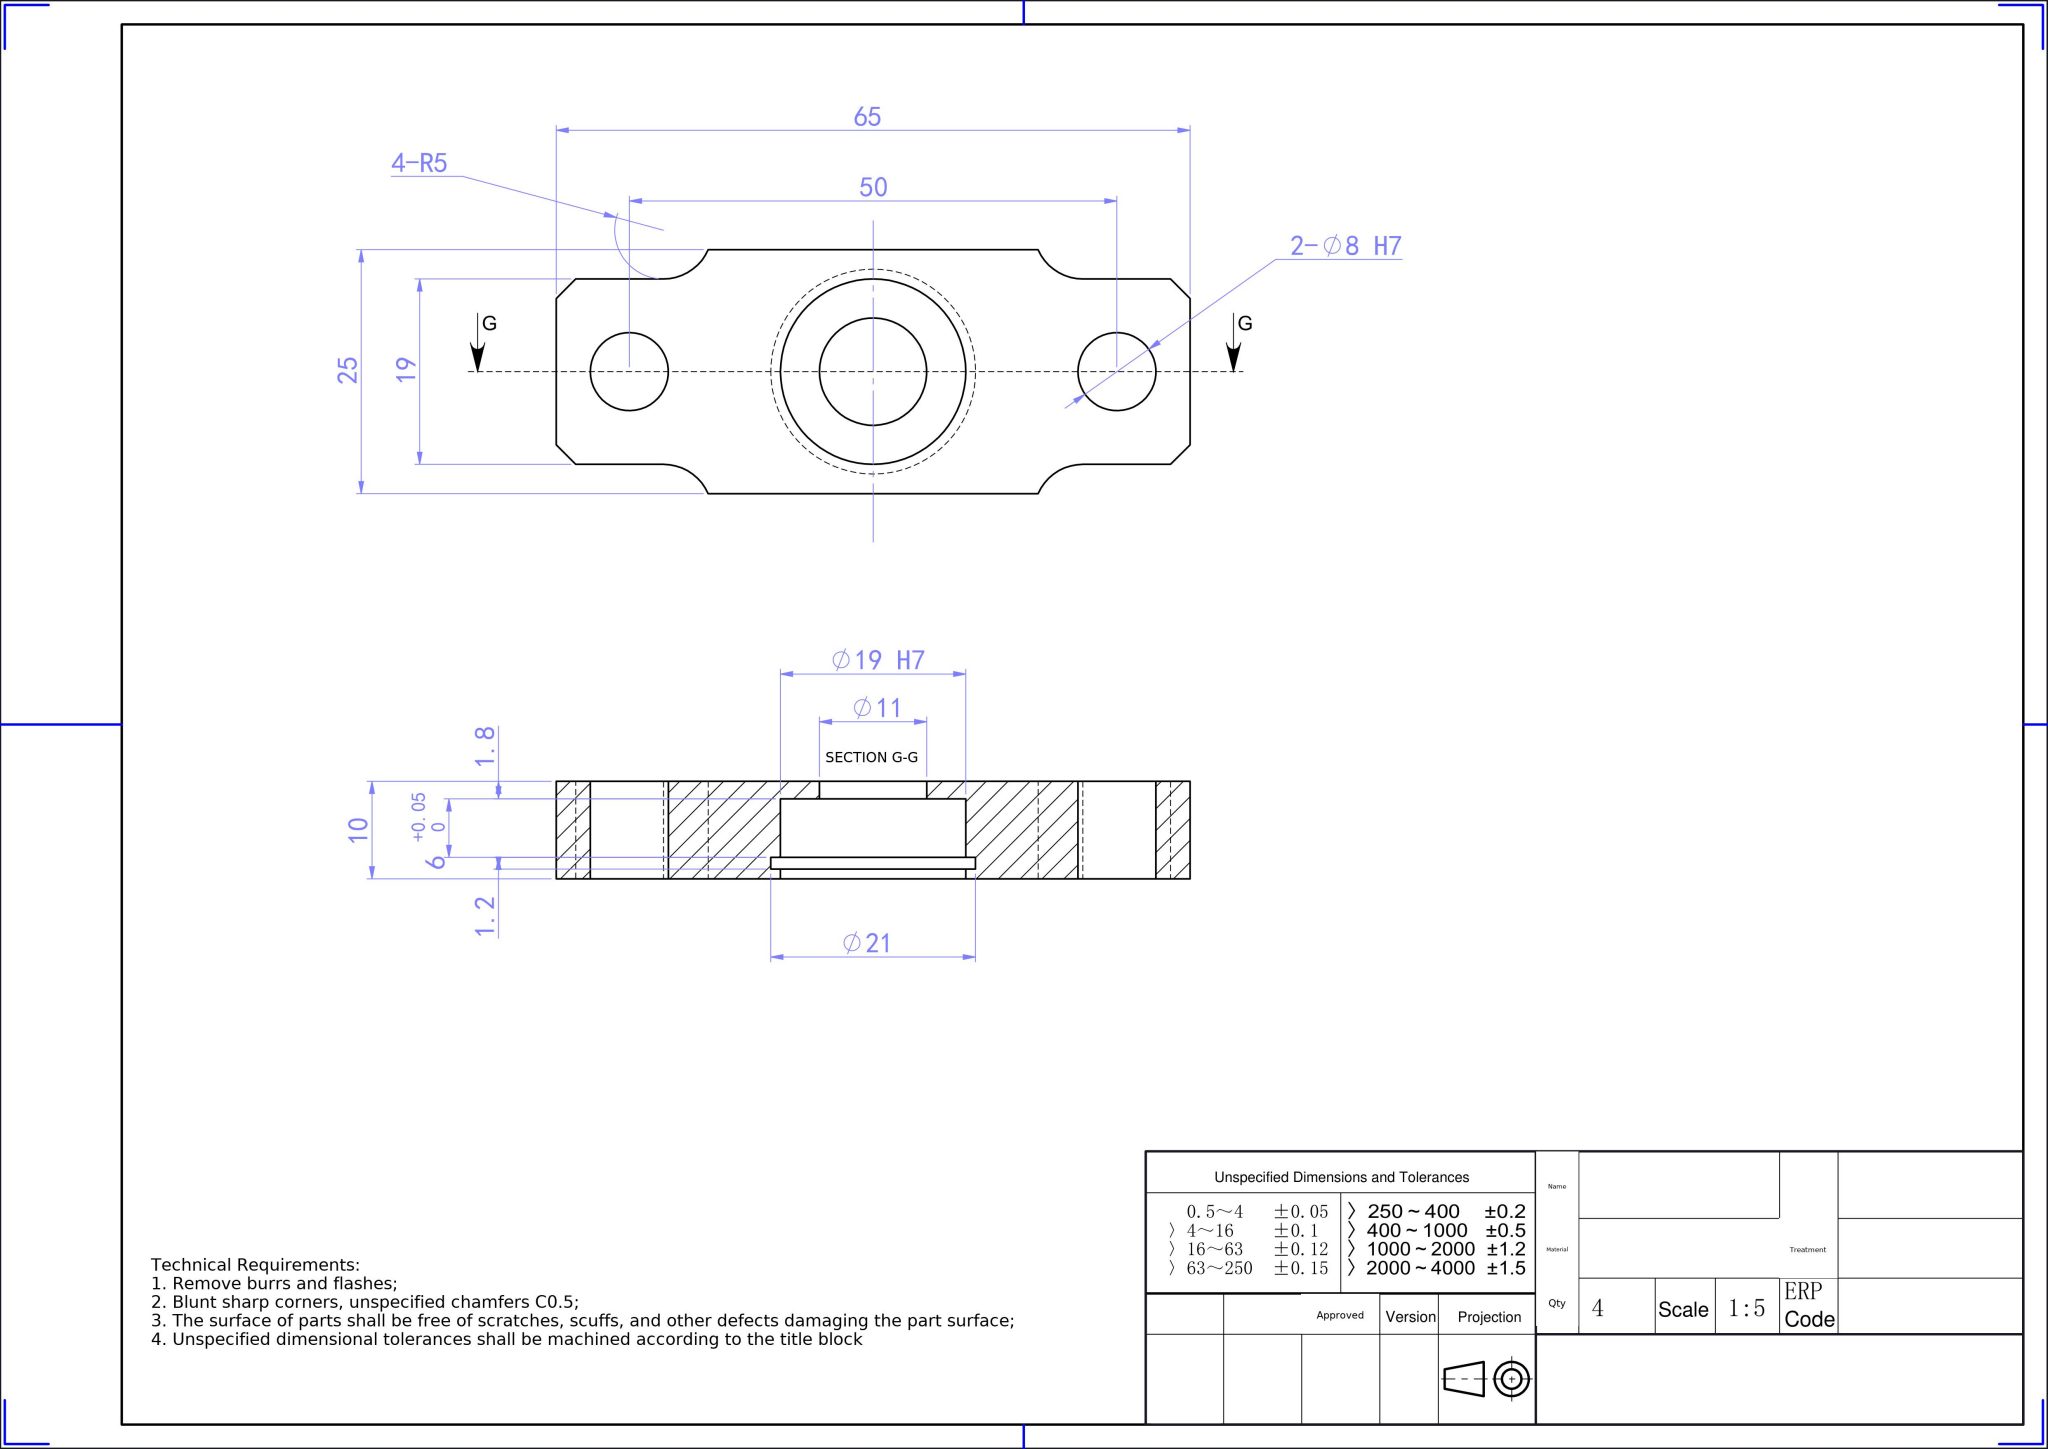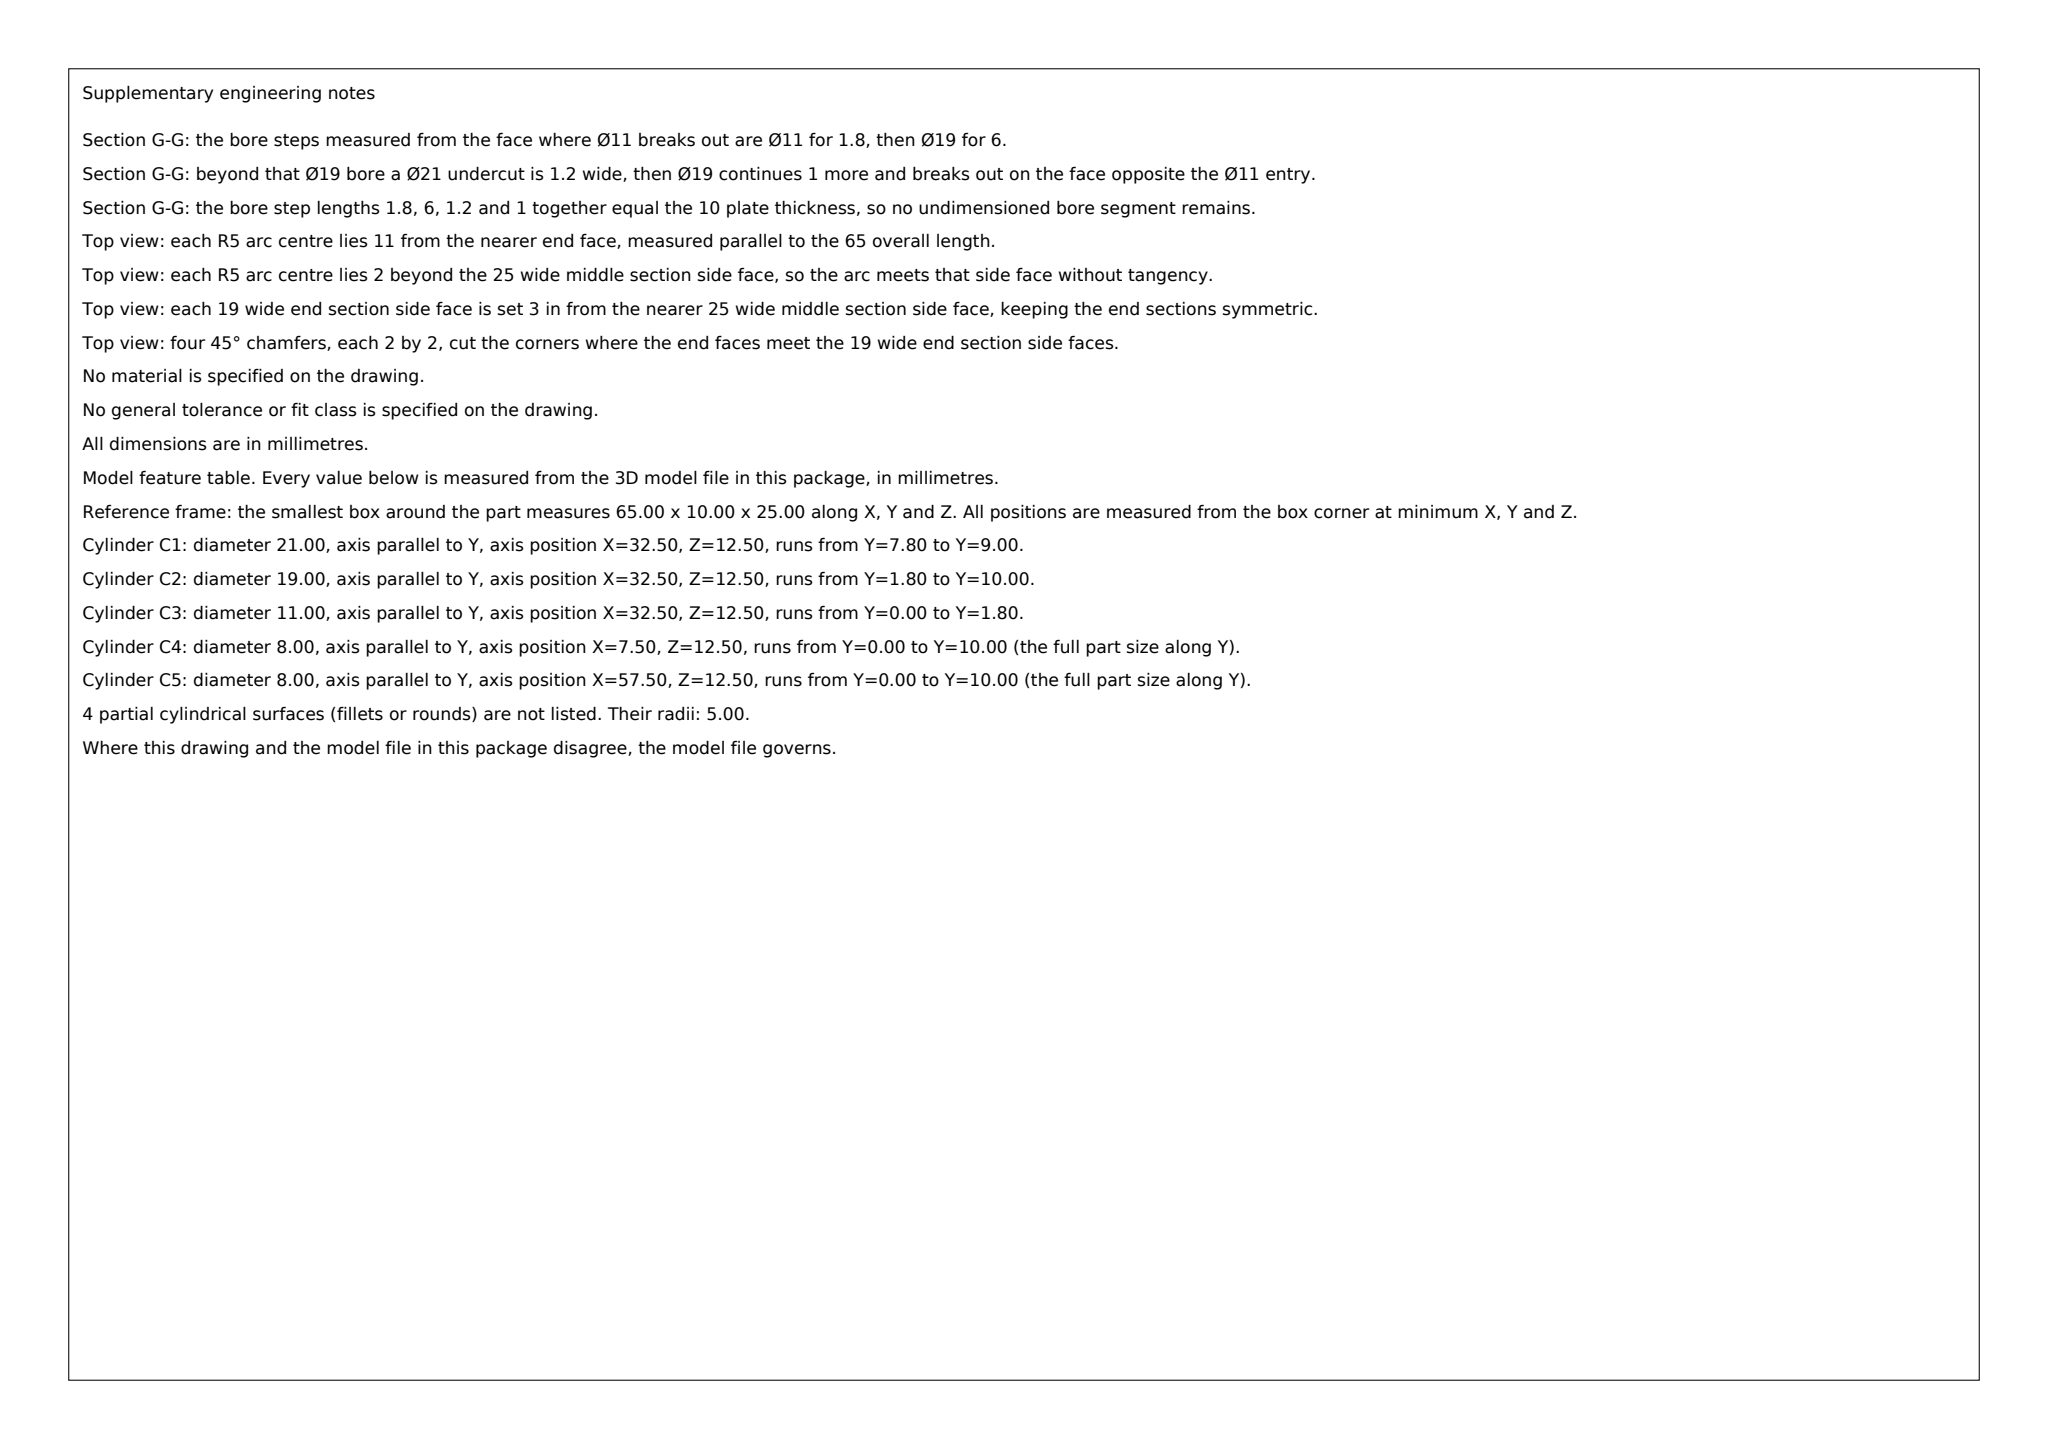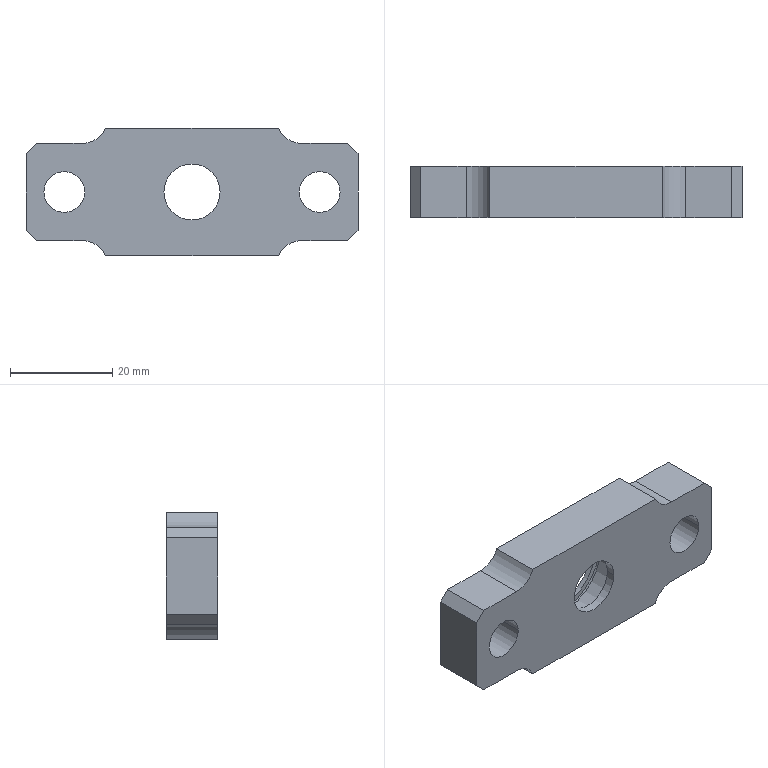Part | SolidWorks | mm | 1 solid | 33 faces | box 65 x 10 x 25 mm | volume 10877 mm3 | plane 17 | cylinder 16 | commonest cylinder face diameters 8 x4 19 x4 10 x4 11 x2 21 x2
Drawing notes:
4-R5 ARC CTRS 11 FROM EA END, 43 APART, ON Ø19 H7 C/L | from the solid: R5 corner cyl dia10 axes at x=11 & x=54 (bbox x=0..65); 65-54=11, 54-11=43; z=-2/27 => tangent to 19 wide flats about z=12.5
build123d program:
from build123d import *

# Parameters (mm, degrees)
SKETCH1_W      = 65
SKETCH1_H      = 10
EXTRUDE1_DEPTH = 25
CHAMFER1_SIZE  = 2
SKETCH11_R     = 4
EXTRUDE3_DEPTH = 18
EXTRUDE4_DEPTH = 18
CHAMFER2_SIZE  = 2


with BuildPart() as part:
    # Sketch1 → Extrude1 (new body)
    with BuildSketch(Plane.XY):
        with Locations((-11.635, 36.458)):
            Rectangle(SKETCH1_W, SKETCH1_H)
    extrude(amount=EXTRUDE1_DEPTH)

    # Chamfer1
    chamfer1_edges = [part.edges().sort_by_distance(p)[0] for p in [
        (20.865, 36.458, 25),
        (-44.135, 36.458, 25),
        (20.865, 36.458, 0),
        (-44.135, 36.458, 0),
    ]]
    chamfer(chamfer1_edges, length=CHAMFER1_SIZE)

    # Sketch9 → Cut-Revolve1 (revolve, cut)
    with BuildSketch(Plane(origin=(0, 0, 12.5), x_dir=(-1, 0, 0), z_dir=(0, 0, -1))):
        Polygon((21.135, 40.458), (22.135, 40.458), (22.135, 39.258), (21.135, 39.258), (21.135, 33.258), (17.135, 33.258), (17.135, 31.458), (11.635, 31.458), (11.635, 41.458), (21.135, 41.458), align=None)
    revolve(axis=Axis((-11.635, 41.458, 12.5), (0, -1, 0)), mode=Mode.SUBTRACT)

    # Sketch11 → Extrude3 (cut)
    with BuildSketch(Plane(origin=(0, 41.458, 0), x_dir=(-1, 0, 0), z_dir=(0, 1, 0))):
        with Locations((36.635, 12.5)):
            Circle(SKETCH11_R)
        with Locations((-13.365, 12.5)):
            Circle(SKETCH11_R)
    extrude(amount=-EXTRUDE3_DEPTH, mode=Mode.SUBTRACT)

    # Sketch12 → Extrude4 (cut)
    with BuildSketch(Plane(origin=(0, 41.458, 0), x_dir=(-1, 0, 0), z_dir=(0, 1, 0))):
        with BuildLine():
            Line((44.135, 22), (44.135, 43.5))
            Line((44.135, 43.5), (28.135, 43.5))
            Line((28.135, 43.5), (28.135, 27))
            ThreePointArc((28.135, 27), (29.599, 23.464), (33.135, 22))
            Line((33.135, 22), (44.135, 22))
        make_face()
        with BuildLine():
            Line((-20.865, 22), (-9.865, 22))
            ThreePointArc((-9.865, 22), (-6.33, 23.464), (-4.865, 27))
            Line((-4.865, 27), (-4.865, 46))
            Line((-4.865, 46), (-20.865, 46))
            Line((-20.865, 46), (-20.865, 22))
        make_face()
        with BuildLine():
            Line((-20.865, 3), (-9.865, 3))
            ThreePointArc((-9.865, 3), (-6.33, 1.536), (-4.865, -2))
            Line((-4.865, -2), (-4.865, -4.365))
            Line((-4.865, -4.365), (-20.865, -4.365))
            Line((-20.865, -4.365), (-20.865, 3))
        make_face()
        with BuildLine():
            Line((44.135, -4.365), (28.135, -4.365))
            Line((28.135, -4.365), (28.135, -2))
            ThreePointArc((28.135, -2), (29.599, 1.536), (33.135, 3))
            Line((33.135, 3), (44.135, 3))
            Line((44.135, 3), (44.135, -4.365))
        make_face()
    extrude(amount=-EXTRUDE4_DEPTH, mode=Mode.SUBTRACT)

    # Chamfer2
    chamfer2_edges = [part.edges().sort_by_distance(p)[0] for p in [
        (20.865, 36.458, 3),
        (-44.135, 36.458, 3),
        (-44.135, 36.458, 22),
        (20.865, 36.458, 22),
    ]]
    chamfer(chamfer2_edges, length=CHAMFER2_SIZE)


solid = part.part